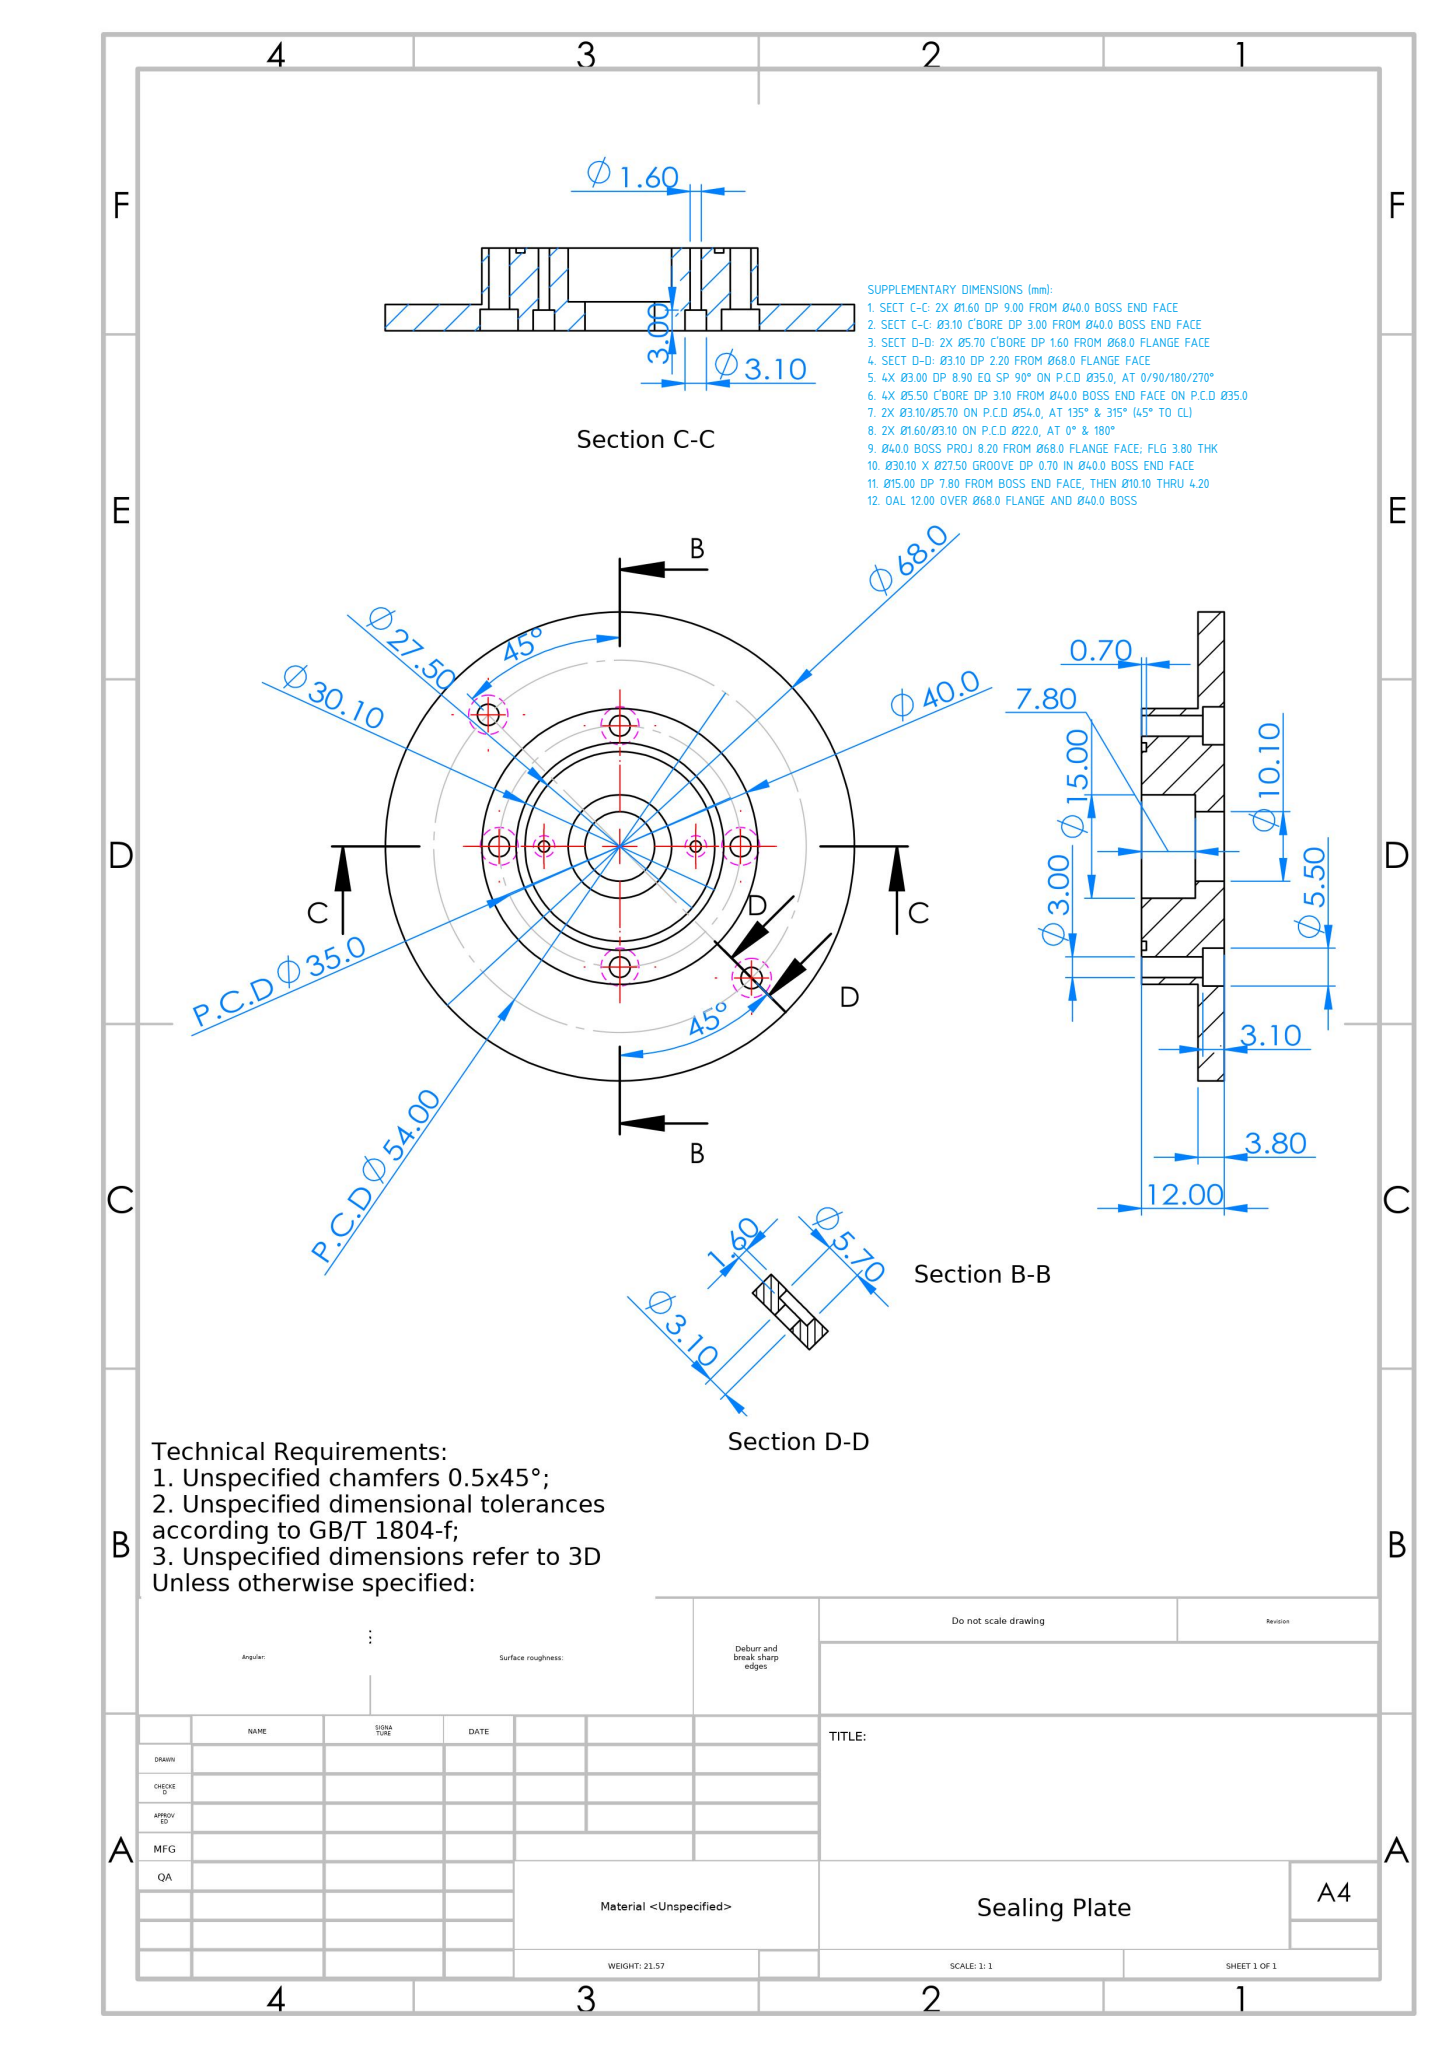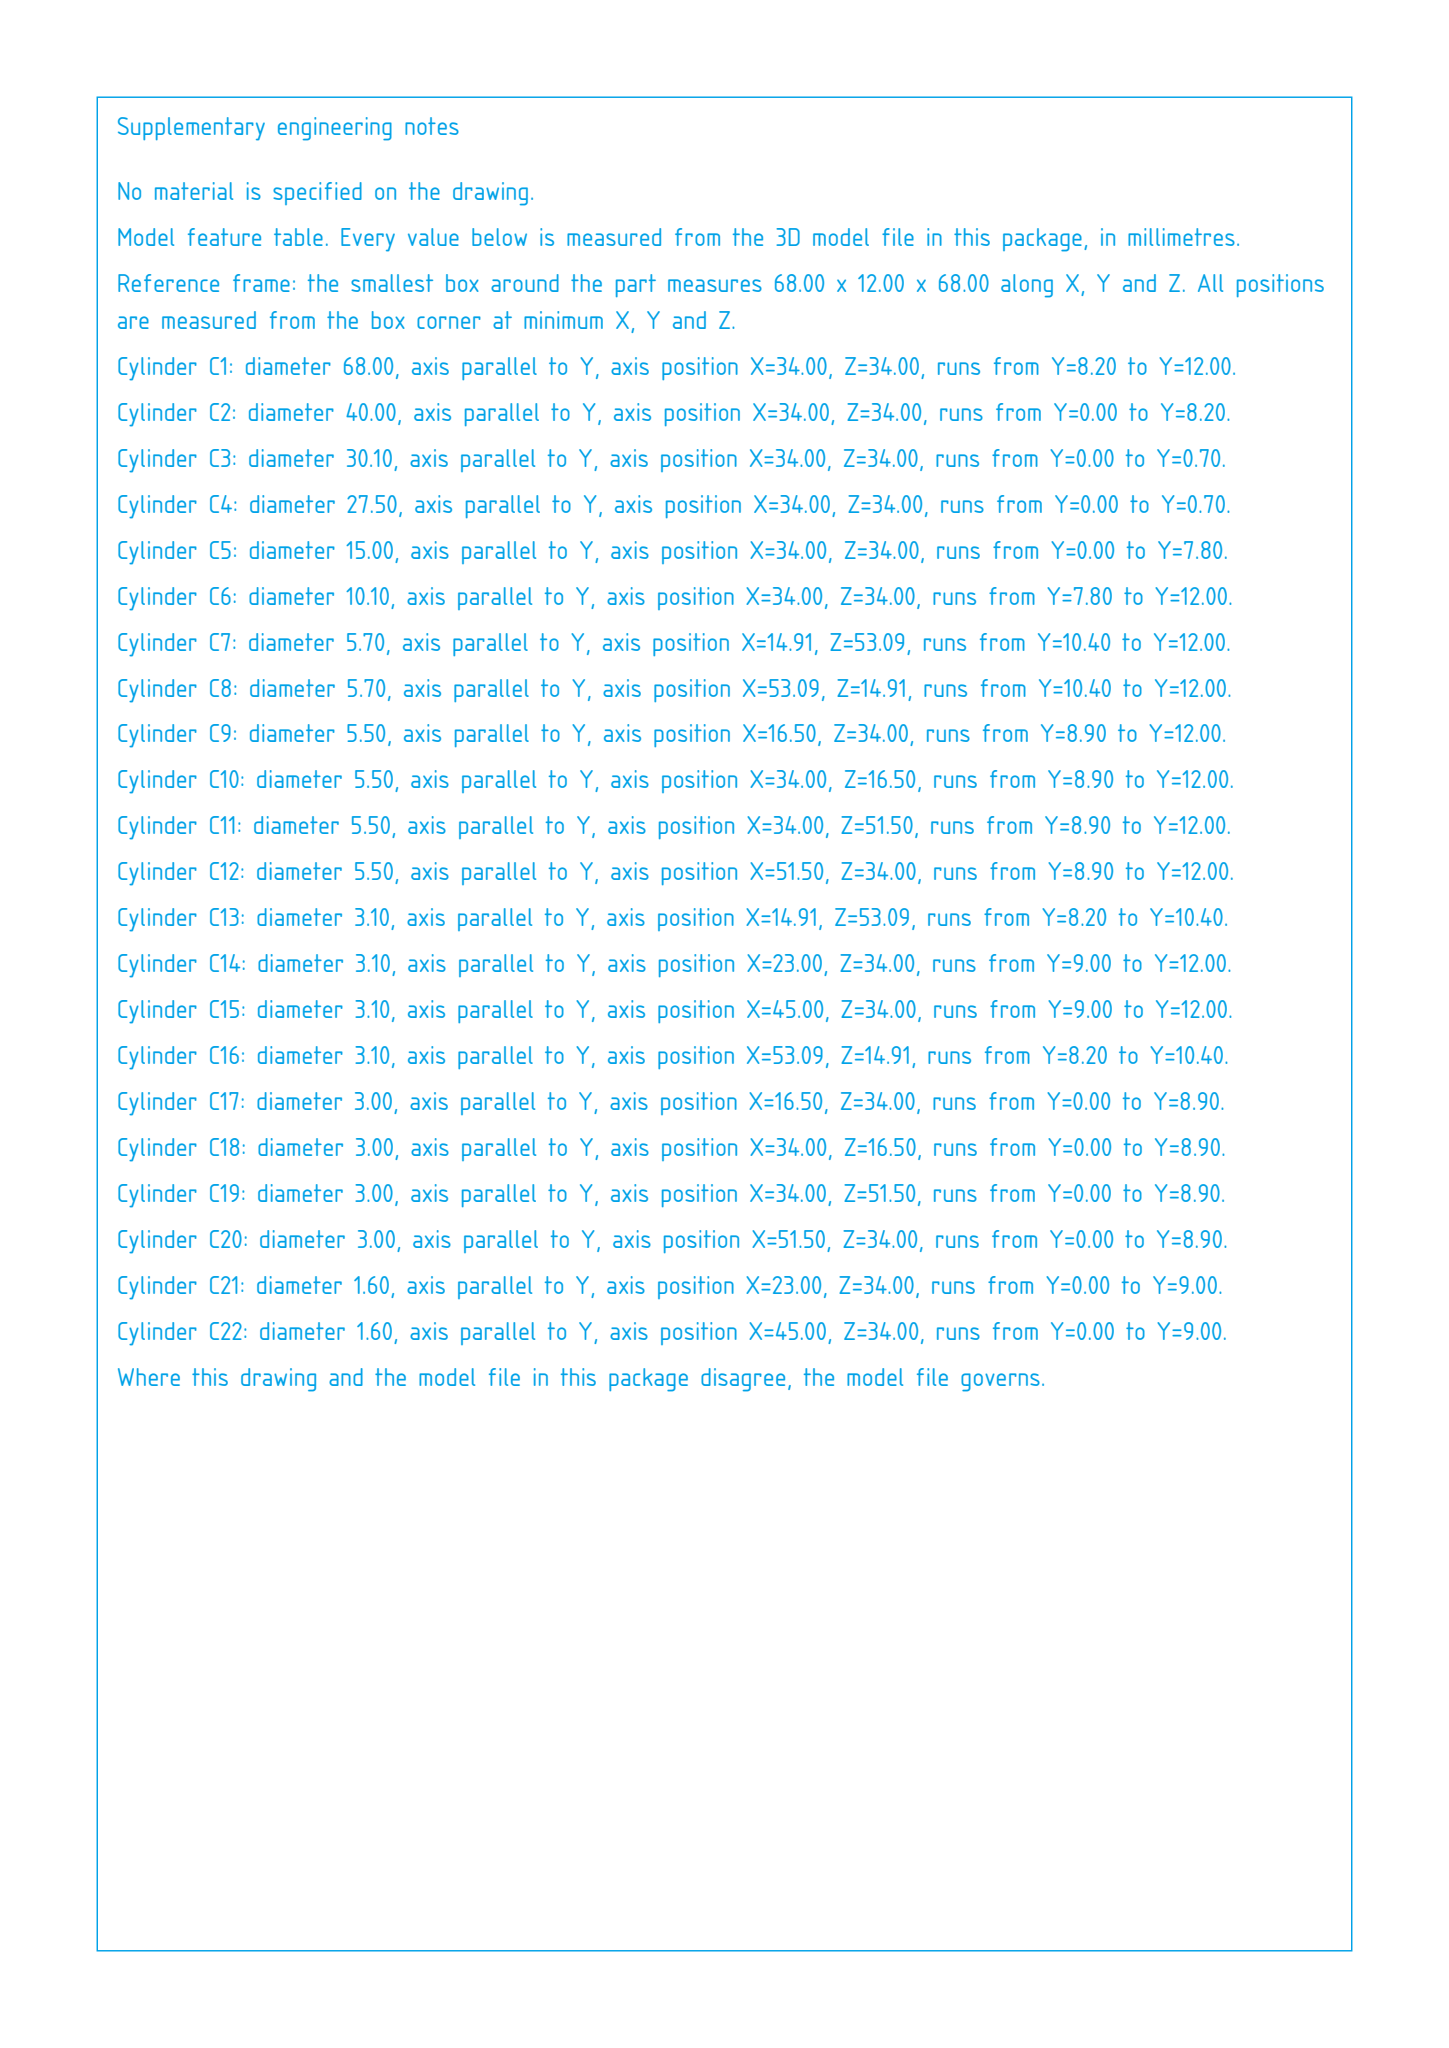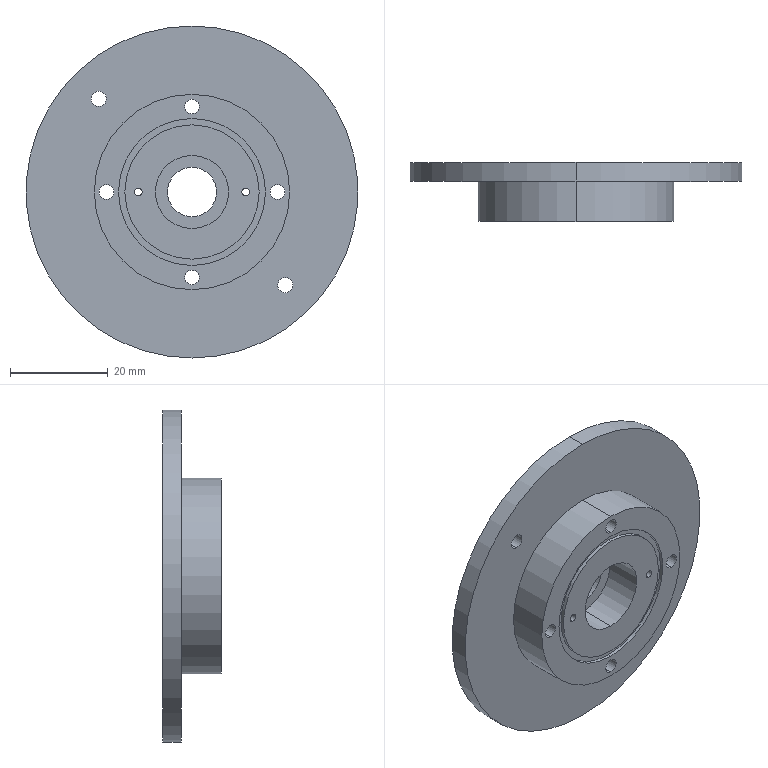Part | SolidWorks | mm | 1 solid | 58 faces | box 68 x 12 x 68 mm | volume 21565 mm3 | cylinder 44 | plane 14 | commonest cylinder face diameters 3 x8 3.1 x8 5.5 x8 5.7 x4 1.6 x4 10.1 x2 68 x2 27.5 x2
build123d program:
from build123d import *

# Parameters (mm, degrees)
SKETCH1_R               = 20
SKETCH1_R_2             = 7.5
BOSS_EXTRUDE1_DEPTH     = 12
SKETCH9_W               = 1.3
SKETCH9_H               = 0.7
SKETCH12_W              = 14
SKETCH12_H              = 3.8
SKETCH5_R               = 0.8
CUT_EXTRUDE2_DEPTH      = 50.558
SKETCH11_R              = 2.75
SKETCH11_R_2            = 1.5
CUT_EXTRUDE4_DEPTH      = 3.1
SKETCH14_W              = 4.95
SKETCH14_H              = 4.2
CUT_EXTRUDE5_DEPTH      = 50.558
CUT_EXTRUDE5_DEPTH_BACK = 1.6
SKETCH15_R              = 2.85
SKETCH7_R               = 1.55
CUT_EXTRUDE3_DEPTH      = 3
SKETCH16_R              = 1.55
CUT_EXTRUDE6_DEPTH      = 50.195
SKETCH17_R              = 1.55
CUT_EXTRUDE7_DEPTH      = 50.195
SKETCH18_R              = 1.5
CUT_EXTRUDE8_DEPTH      = 50.558


with BuildPart() as part:
    # Sketch1 → Boss-Extrude1 (new body)
    with BuildSketch(Plane(origin=(0, 0, 0), x_dir=(1, 0, 0), z_dir=(0, 1, 0))):
        with Locations(Location((0, 0, 0), (0, 0, 270))):
            Circle(SKETCH1_R)
        with Locations(Location((0, 0, 0), (0, 0, 270))):
            Circle(SKETCH1_R_2, mode=Mode.SUBTRACT)
    extrude(amount=BOSS_EXTRUDE1_DEPTH)

    # Sketch9 → Cut-Revolve3 (revolve, cut)
    with BuildSketch(Plane.XY, mode=Mode.PRIVATE) as cut_revolve3_sk:
        with Locations((14.4, 0.35)):
            Rectangle(SKETCH9_W, SKETCH9_H)
    revolve(cut_revolve3_sk.sketch.rotate(Axis((0, -3.122, 0), (0, 1, 0)), 90), axis=Axis((0, -3.122, 0), (0, 1, 0)), mode=Mode.SUBTRACT)

    # Sketch12 → Revolve1 (revolve)
    with BuildSketch(Plane.XY, mode=Mode.PRIVATE) as revolve1_sk:
        with Locations((27, 10.1)):
            Rectangle(SKETCH12_W, SKETCH12_H)
    revolve(revolve1_sk.sketch.rotate(Axis((0, 0, 0), (0, 1, 0)), 90), axis=Axis((0, 0, 0), (0, 1, 0)))

    # Sketch5 → Cut-Extrude2 (cut, through all)
    with BuildSketch(Plane(origin=(0, 12, 0), x_dir=(1, 0, 0), z_dir=(0, 1, 0))):
        with Locations(Location((11, 0, 0), (0, 0, 270))):
            Circle(SKETCH5_R)
        with Locations(Location((-11, 0, 0), (0, 0, 270))):
            Circle(SKETCH5_R)
    extrude(amount=-CUT_EXTRUDE2_DEPTH, mode=Mode.SUBTRACT)

    # Sketch11 → Cut-Extrude4 (cut)
    # profile 1 of 4: a face of its own
    with BuildSketch(Plane(origin=(0, 12, 0), x_dir=(1, 0, 0), z_dir=(0, 1, 0))):
        with Locations(Location((-17.5, 0, 0), (0, 0, 270))):
            Circle(SKETCH11_R)
        with Locations(Location((-17.5, 0, 0), (0, 0, 270))):
            Circle(SKETCH11_R_2, mode=Mode.SUBTRACT)
    # profile 2 of 4: a face of its own
    with BuildSketch(Plane(origin=(0, 12, 0), x_dir=(1, 0, 0), z_dir=(0, 1, 0))):
        with Locations(Location((0, 17.5, 0), (0, 0, 270))):
            Circle(SKETCH11_R)
        with Locations(Location((0, 17.5, 0), (0, 0, 270))):
            Circle(SKETCH11_R_2, mode=Mode.SUBTRACT)
    # profile 3 of 4: a face of its own
    with BuildSketch(Plane(origin=(0, 12, 0), x_dir=(1, 0, 0), z_dir=(0, 1, 0))):
        with Locations(Location((17.5, 0, 0), (0, 0, 270))):
            Circle(SKETCH11_R)
        with Locations(Location((17.5, 0, 0), (0, 0, 270))):
            Circle(SKETCH11_R_2, mode=Mode.SUBTRACT)
    # profile 4 of 4: a face of its own
    with BuildSketch(Plane(origin=(0, 12, 0), x_dir=(1, 0, 0), z_dir=(0, 1, 0))):
        with Locations(Location((0, -17.5, 0), (0, 0, 270))):
            Circle(SKETCH11_R)
        with Locations(Location((0, -17.5, 0), (0, 0, 270))):
            Circle(SKETCH11_R_2, mode=Mode.SUBTRACT)
    extrude(amount=-CUT_EXTRUDE4_DEPTH, mode=Mode.SUBTRACT)

    # Sketch14 → Revolve2 (revolve)
    with BuildSketch(Plane.XY, mode=Mode.PRIVATE) as revolve2_sk:
        with Locations((7.525, 9.9)):
            Rectangle(SKETCH14_W, SKETCH14_H)
    revolve(revolve2_sk.sketch.rotate(Axis((0, -21.996, 0), (0, 1, 0)), 90), axis=Axis((0, -21.996, 0), (0, 1, 0)))

    # Sketch15 → Cut-Extrude5 (cut, two sides: drawn at the far end of the back side and taken through both)
    with BuildSketch(Plane(origin=(0, 12, 0), x_dir=(1, 0, 0), z_dir=(0, 1, 0)).offset(-CUT_EXTRUDE5_DEPTH_BACK)):
        with Locations(Location((-19.092, -19.092, 0), (0, 0, 90))):
            Circle(SKETCH15_R)
        with Locations(Location((19.092, 19.092, 0), (0, 0, 90))):
            Circle(SKETCH15_R)
    extrude(amount=CUT_EXTRUDE5_DEPTH + CUT_EXTRUDE5_DEPTH_BACK, mode=Mode.SUBTRACT)

    # Sketch7 → Cut-Extrude3 (cut)
    with BuildSketch(Plane(origin=(0, 12, 0), x_dir=(1, 0, 0), z_dir=(0, 1, 0))):
        with Locations(Location((11, 0, 0), (0, 0, 270))):
            Circle(SKETCH7_R)
        with Locations(Location((-11, 0, 0), (0, 0, 270))):
            Circle(SKETCH7_R)
    extrude(amount=-CUT_EXTRUDE3_DEPTH, mode=Mode.SUBTRACT)

    # Sketch16 → Cut-Extrude6 (cut, through all)
    with BuildSketch(Plane(origin=(0, 10.4, 0), x_dir=(1, 0, 0), z_dir=(0, 1, 0))):
        with Locations(Location((-19.092, -19.092, 0), (0, 0, 270))):
            Circle(SKETCH16_R)
    extrude(amount=-CUT_EXTRUDE6_DEPTH, mode=Mode.SUBTRACT)

    # Sketch17 → Cut-Extrude7 (cut, through all)
    with BuildSketch(Plane(origin=(0, 10.4, 0), x_dir=(1, 0, 0), z_dir=(0, 1, 0))):
        with Locations(Location((19.092, 19.092, 0), (0, 0, 270))):
            Circle(SKETCH17_R)
    extrude(amount=-CUT_EXTRUDE7_DEPTH, mode=Mode.SUBTRACT)

    # Sketch18 → Cut-Extrude8 (cut, through all)
    with BuildSketch(Plane(origin=(0, 12, 0), x_dir=(1, 0, 0), z_dir=(0, 1, 0))):
        with Locations(Location((0, 17.5, 0), (0, 0, 270))):
            Circle(SKETCH18_R)
        with Locations(Location((-17.5, 0, 0), (0, 0, 270))):
            Circle(SKETCH18_R)
        with Locations(Location((0, -17.5, 0), (0, 0, 270))):
            Circle(SKETCH18_R)
        with Locations(Location((17.5, 0, 0), (0, 0, 270))):
            Circle(SKETCH18_R)
    extrude(amount=-CUT_EXTRUDE8_DEPTH, mode=Mode.SUBTRACT)


solid = part.part